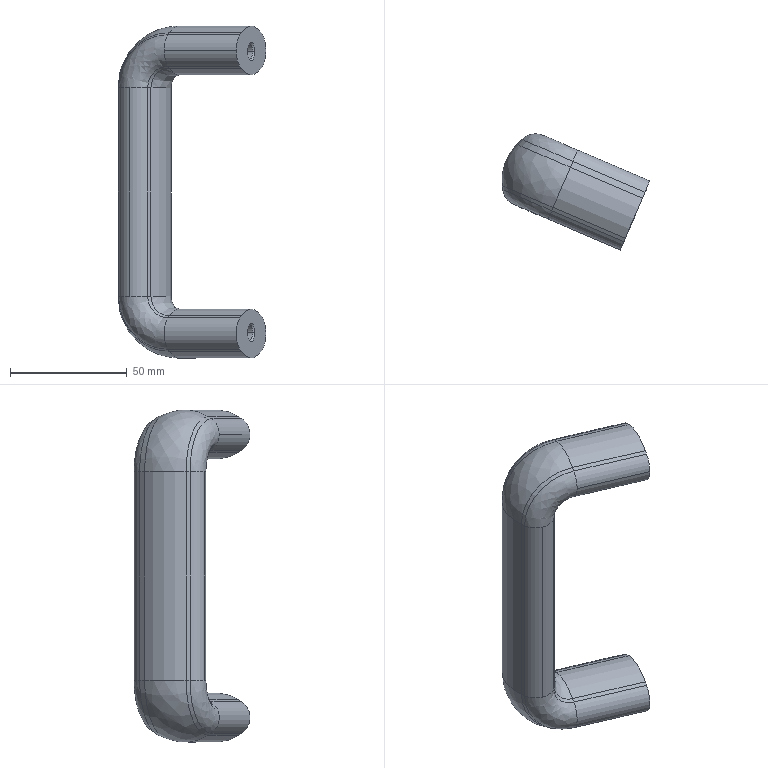Component | SolidWorks | UPCFN120Handle-2 | 1 solid | 57 faces | volume 106957 mm3 | cylinder 19 | cone 16 | plane 14 | spline 8 | commonest cylinder face diameters 42 x6 15.54 x5 16.8 x4 6.647 x4